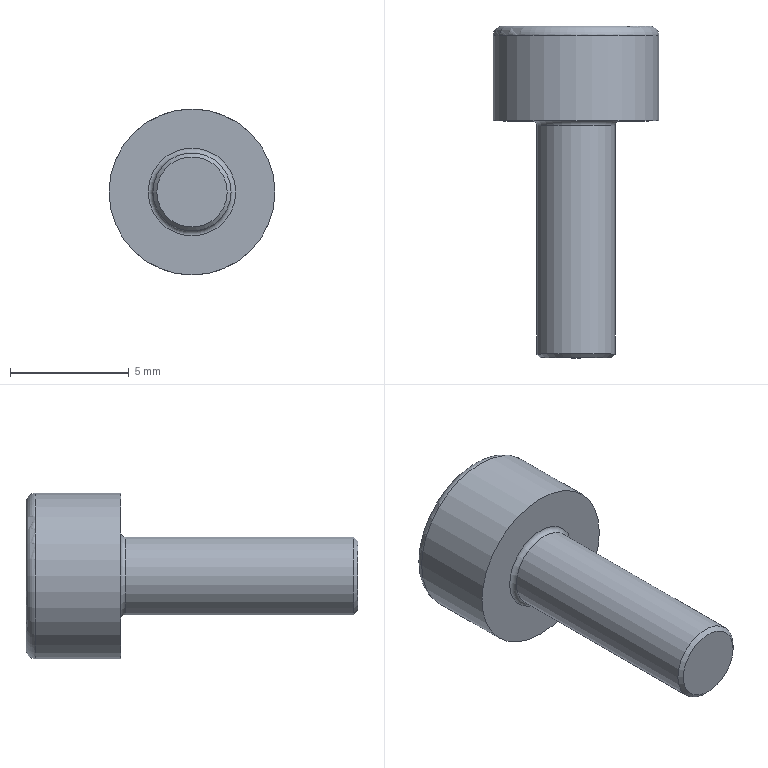Component | NX | SCREW_M4X10 | 1 solid | 27 faces | volume 216 mm3 | plane 15 | cone 8 | cylinder 2 | torus 2 | commonest cylinder face diameters 3.3 x1 7 x1